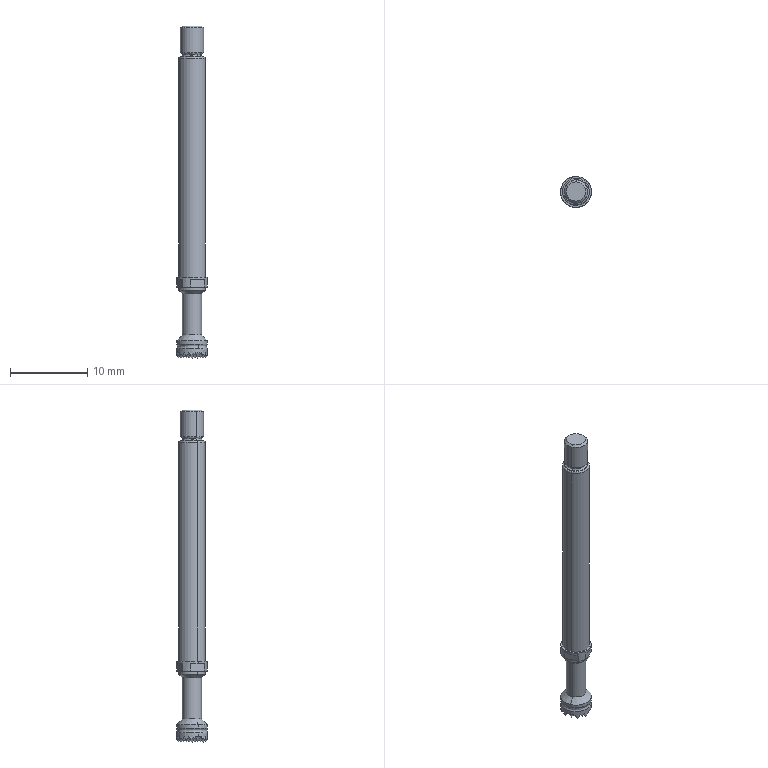Component | SolidWorks | 170423A4-INGUN HSS150-1_170423A4-INGUN_HSS-150_306_400_02_M-1 | 1 solid | 207 faces | box 4 x 4 x 43.1 mm | volume 379 mm3 | plane 145 | spline 30 | cylinder 26 | cone 6 | commonest cylinder face diameters 2.5 x8 4 x6 2.4 x6 3.5 x2 3.48 x2 3 x2